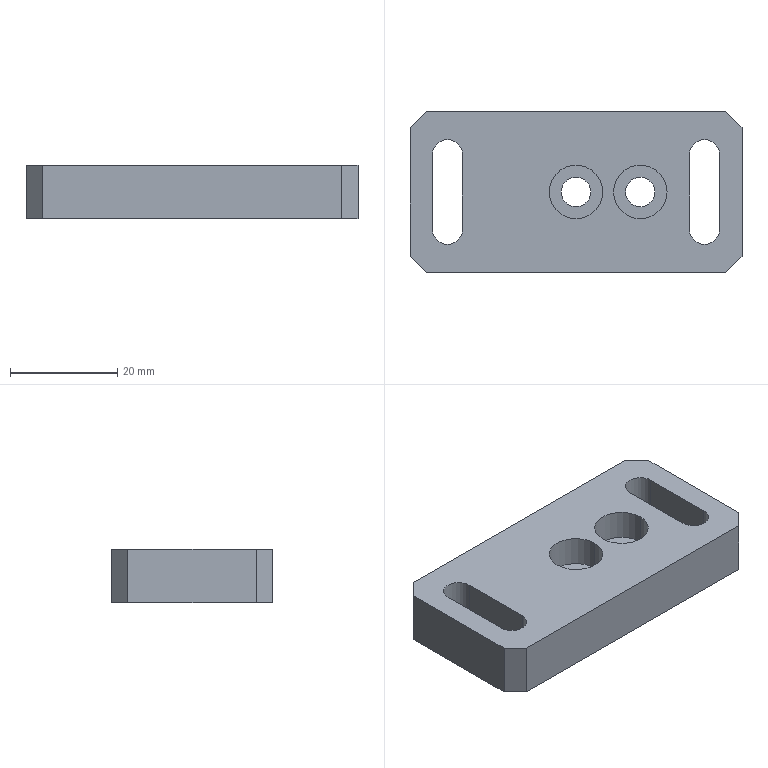Component | SolidWorks | A52-1 | 1 solid | 28 faces | box 62 x 30 x 10 mm | volume 15260 mm3 | plane 16 | cylinder 12 | commonest cylinder face diameters 10 x4 5.5 x4 5.6 x4 | material A6061
build123d program:
from build123d import *

# Parameters (mm, degrees)
SKETCH1_W                                         = 62
SKETCH1_H                                         = 30
BOSS_EXTRUDE1_DEPTH                               = 5
CHAMFER1_SIZE                                     = 3
CUT_EXTRUDE1_DEPTH                                = 36.861
HOLE_SIZE_ACCORDING_TO_HEXAGON_SOCKET_D           = 5.5
HOLE_SIZE_ACCORDING_TO_HEXAGON_SOCKET_CBORE_D     = 10
HOLE_SIZE_ACCORDING_TO_HEXAGON_SOCKET_CBORE_DEPTH = 5.7


with BuildPart() as part:
    # Sketch1 → Boss-Extrude1 (new, symmetric)
    with BuildSketch(Plane(origin=(0, 0, 0), x_dir=(0, 0, -1), z_dir=(1, 0, 0))):
        Rectangle(SKETCH1_W, SKETCH1_H)
    extrude(amount=BOSS_EXTRUDE1_DEPTH, both=True)

    # Chamfer1
    chamfer1_edges = [part.edges().sort_by_distance(p)[0] for p in [
        (0, -15, -31),
        (0, -15, 31),
        (0, 15, 31),
        (0, 15, -31),
    ]]
    chamfer(chamfer1_edges, length=CHAMFER1_SIZE)

    # Sketch2 → Cut-Extrude1 (cut, through all)
    with BuildSketch(Plane.ZY.offset(5)):
        with BuildLine():
            Line((-21.2, 7), (-21.2, -7))
            ThreePointArc((-21.2, -7), (-24, -9.8), (-26.8, -7))
            Line((-26.8, -7), (-26.8, 7))
            ThreePointArc((-26.8, 7), (-24, 9.8), (-21.2, 7))
        make_face()
        with BuildLine():
            Line((26.8, 7), (26.8, -7))
            ThreePointArc((26.8, -7), (24, -9.8), (21.2, -7))
            Line((21.2, -7), (21.2, 7))
            ThreePointArc((21.2, 7), (24, 9.8), (26.8, 7))
        make_face()
    extrude(amount=-CUT_EXTRUDE1_DEPTH, mode=Mode.SUBTRACT)

    # Hole Size _according to_ Hexagon Socket (through all)
    with Locations(Plane(origin=(5, 0, 0), x_dir=(0, 0, -1), z_dir=(1, 0, 0))):
        with Locations((0, 0), (12, 0)):
            CounterBoreHole(HOLE_SIZE_ACCORDING_TO_HEXAGON_SOCKET_D / 2, HOLE_SIZE_ACCORDING_TO_HEXAGON_SOCKET_CBORE_D / 2, HOLE_SIZE_ACCORDING_TO_HEXAGON_SOCKET_CBORE_DEPTH)


solid = part.part

# Placed as in the assembly
solid = solid.moved(Location((-12.351, 25.864, 35), (0, -90, 0)))
STEP:
#1=COLOUR_RGB('',0.7922,0.8196,0.9333);
#2=FILL_AREA_STYLE_COLOUR('',#1);
#3=FILL_AREA_STYLE('',(#2));
#4=SURFACE_STYLE_FILL_AREA(#3);
#5=SURFACE_SIDE_STYLE('',(#4));
#6=SURFACE_STYLE_USAGE(.BOTH.,#5);
#7=PRESENTATION_STYLE_ASSIGNMENT((#6));
#8=CARTESIAN_POINT('',(-0.6831,1.018,1.35));
#9=VERTEX_POINT('',#8);
#10=CARTESIAN_POINT('',(-0.2894,1.018,1.35));
#11=VERTEX_POINT('',#10);
#12=CARTESIAN_POINT('',(-0.4863,1.018,1.35));
#13=DIRECTION('',(0.,0.,1.));
#14=DIRECTION('',(1.,0.,0.));
#15=AXIS2_PLACEMENT_3D('',#12,#13,#14);
#16=CIRCLE('',#15,0.1969);
#17=EDGE_CURVE('',#9,#11,#16,.T.);
#18=ORIENTED_EDGE('',*,*,#17,.F.);
#19=CARTESIAN_POINT('',(-0.6831,1.018,1.575));
#20=VERTEX_POINT('',#19);
#21=CARTESIAN_POINT('',(-0.6831,1.018,1.575));
#22=DIRECTION('',(0.,0.,1.));
#23=VECTOR('',#22,39.37);
#24=LINE('',#21,#23);
#25=EDGE_CURVE('',#9,#20,#24,.T.);
#26=ORIENTED_EDGE('',*,*,#25,.T.);
#27=CARTESIAN_POINT('',(-0.2894,1.018,1.575));
#28=VERTEX_POINT('',#27);
#29=CARTESIAN_POINT('',(-0.4863,1.018,1.575));
#30=DIRECTION('',(0.,0.,1.));
#31=DIRECTION('',(1.,0.,0.));
#32=AXIS2_PLACEMENT_3D('',#29,#30,#31);
#33=CIRCLE('',#32,0.1969);
#34=EDGE_CURVE('',#20,#28,#33,.T.);
#35=ORIENTED_EDGE('',*,*,#34,.T.);
#36=CARTESIAN_POINT('',(-0.2894,1.018,1.575));
#37=DIRECTION('',(0.,0.,1.));
#38=VECTOR('',#37,39.37);
#39=LINE('',#36,#38);
#40=EDGE_CURVE('',#11,#28,#39,.T.);
#41=ORIENTED_EDGE('',*,*,#40,.F.);
#42=EDGE_LOOP('',(#18,#26,#35,#41));
#43=FACE_OUTER_BOUND('',#42,.T.);
#44=CARTESIAN_POINT('',(-0.4863,1.018,1.575));
#45=DIRECTION('',(0.,0.,1.));
#46=DIRECTION('',(1.,0.,0.));
#47=AXIS2_PLACEMENT_3D('',#44,#45,#46);
#48=CYLINDRICAL_SURFACE('',#47,0.1969);
#49=ADVANCED_FACE('',(#43),#48,.F.);
#50=CARTESIAN_POINT('',(-0.5945,1.018,1.181));
#51=VERTEX_POINT('',#50);
#52=CARTESIAN_POINT('',(-0.378,1.018,1.181));
#53=VERTEX_POINT('',#52);
#54=CARTESIAN_POINT('',(-0.4863,1.018,1.181));
#55=DIRECTION('',(0.,0.,1.));
#56=DIRECTION('',(1.,0.,0.));
#57=AXIS2_PLACEMENT_3D('',#54,#55,#56);
#58=CIRCLE('',#57,0.1083);
#59=EDGE_CURVE('',#51,#53,#58,.T.);
#60=ORIENTED_EDGE('',*,*,#59,.F.);
#61=CARTESIAN_POINT('',(-0.5945,1.018,1.35));
#62=VERTEX_POINT('',#61);
#63=CARTESIAN_POINT('',(-0.5945,1.018,1.575));
#64=DIRECTION('',(0.,0.,1.));
#65=VECTOR('',#64,39.37);
#66=LINE('',#63,#65);
#67=EDGE_CURVE('',#51,#62,#66,.T.);
#68=ORIENTED_EDGE('',*,*,#67,.T.);
#69=CARTESIAN_POINT('',(-0.378,1.018,1.35));
#70=VERTEX_POINT('',#69);
#71=CARTESIAN_POINT('',(-0.4863,1.018,1.35));
#72=DIRECTION('',(0.,0.,1.));
#73=DIRECTION('',(1.,0.,0.));
#74=AXIS2_PLACEMENT_3D('',#71,#72,#73);
#75=CIRCLE('',#74,0.1083);
#76=EDGE_CURVE('',#62,#70,#75,.T.);
#77=ORIENTED_EDGE('',*,*,#76,.T.);
#78=CARTESIAN_POINT('',(-0.378,1.018,1.575));
#79=DIRECTION('',(0.,0.,1.));
#80=VECTOR('',#79,39.37);
#81=LINE('',#78,#80);
#82=EDGE_CURVE('',#53,#70,#81,.T.);
#83=ORIENTED_EDGE('',*,*,#82,.F.);
#84=EDGE_LOOP('',(#60,#68,#77,#83));
#85=FACE_OUTER_BOUND('',#84,.T.);
#86=CARTESIAN_POINT('',(-0.4863,1.018,1.575));
#87=DIRECTION('',(0.,0.,1.));
#88=DIRECTION('',(1.,0.,0.));
#89=AXIS2_PLACEMENT_3D('',#86,#87,#88);
#90=CYLINDRICAL_SURFACE('',#89,0.1083);
#91=ADVANCED_FACE('',(#85),#90,.F.);
#92=CARTESIAN_POINT('',(-0.2107,1.018,1.35));
#93=VERTEX_POINT('',#92);
#94=CARTESIAN_POINT('',(0.183,1.018,1.35));
#95=VERTEX_POINT('',#94);
#96=CARTESIAN_POINT('',(-0.01381,1.018,1.35));
#97=DIRECTION('',(0.,0.,1.));
#98=DIRECTION('',(1.,0.,0.));
#99=AXIS2_PLACEMENT_3D('',#96,#97,#98);
#100=CIRCLE('',#99,0.1969);
#101=EDGE_CURVE('',#93,#95,#100,.T.);
#102=ORIENTED_EDGE('',*,*,#101,.F.);
#103=CARTESIAN_POINT('',(-0.2107,1.018,1.575));
#104=VERTEX_POINT('',#103);
#105=CARTESIAN_POINT('',(-0.2107,1.018,1.575));
#106=DIRECTION('',(0.,0.,1.));
#107=VECTOR('',#106,39.37);
#108=LINE('',#105,#107);
#109=EDGE_CURVE('',#93,#104,#108,.T.);
#110=ORIENTED_EDGE('',*,*,#109,.T.);
#111=CARTESIAN_POINT('',(0.183,1.018,1.575));
#112=VERTEX_POINT('',#111);
#113=CARTESIAN_POINT('',(-0.01381,1.018,1.575));
#114=DIRECTION('',(0.,0.,1.));
#115=DIRECTION('',(1.,0.,0.));
#116=AXIS2_PLACEMENT_3D('',#113,#114,#115);
#117=CIRCLE('',#116,0.1969);
#118=EDGE_CURVE('',#104,#112,#117,.T.);
#119=ORIENTED_EDGE('',*,*,#118,.T.);
#120=CARTESIAN_POINT('',(0.183,1.018,1.575));
#121=DIRECTION('',(0.,0.,1.));
#122=VECTOR('',#121,39.37);
#123=LINE('',#120,#122);
#124=EDGE_CURVE('',#95,#112,#123,.T.);
#125=ORIENTED_EDGE('',*,*,#124,.F.);
#126=EDGE_LOOP('',(#102,#110,#119,#125));
#127=FACE_OUTER_BOUND('',#126,.T.);
#128=CARTESIAN_POINT('',(-0.01381,1.018,1.575));
#129=DIRECTION('',(0.,0.,1.));
#130=DIRECTION('',(1.,0.,0.));
#131=AXIS2_PLACEMENT_3D('',#128,#129,#130);
#132=CYLINDRICAL_SURFACE('',#131,0.1969);
#133=ADVANCED_FACE('',(#127),#132,.F.);
#134=CARTESIAN_POINT('',(-0.1221,1.018,1.181));
#135=VERTEX_POINT('',#134);
#136=CARTESIAN_POINT('',(0.09446,1.018,1.181));
#137=VERTEX_POINT('',#136);
#138=CARTESIAN_POINT('',(-0.01381,1.018,1.181));
#139=DIRECTION('',(0.,0.,1.));
#140=DIRECTION('',(1.,0.,0.));
#141=AXIS2_PLACEMENT_3D('',#138,#139,#140);
#142=CIRCLE('',#141,0.1083);
#143=EDGE_CURVE('',#135,#137,#142,.T.);
#144=ORIENTED_EDGE('',*,*,#143,.F.);
#145=CARTESIAN_POINT('',(-0.1221,1.018,1.35));
#146=VERTEX_POINT('',#145);
#147=CARTESIAN_POINT('',(-0.1221,1.018,1.575));
#148=DIRECTION('',(0.,0.,1.));
#149=VECTOR('',#148,39.37);
#150=LINE('',#147,#149);
#151=EDGE_CURVE('',#135,#146,#150,.T.);
#152=ORIENTED_EDGE('',*,*,#151,.T.);
#153=CARTESIAN_POINT('',(0.09446,1.018,1.35));
#154=VERTEX_POINT('',#153);
#155=CARTESIAN_POINT('',(-0.01381,1.018,1.35));
#156=DIRECTION('',(0.,0.,1.));
#157=DIRECTION('',(1.,0.,0.));
#158=AXIS2_PLACEMENT_3D('',#155,#156,#157);
#159=CIRCLE('',#158,0.1083);
#160=EDGE_CURVE('',#146,#154,#159,.T.);
#161=ORIENTED_EDGE('',*,*,#160,.T.);
#162=CARTESIAN_POINT('',(0.09446,1.018,1.575));
#163=DIRECTION('',(0.,0.,1.));
#164=VECTOR('',#163,39.37);
#165=LINE('',#162,#164);
#166=EDGE_CURVE('',#137,#154,#165,.T.);
#167=ORIENTED_EDGE('',*,*,#166,.F.);
#168=EDGE_LOOP('',(#144,#152,#161,#167));
#169=FACE_OUTER_BOUND('',#168,.T.);
#170=CARTESIAN_POINT('',(-0.01381,1.018,1.575));
#171=DIRECTION('',(0.,0.,1.));
#172=DIRECTION('',(1.,0.,0.));
#173=AXIS2_PLACEMENT_3D('',#170,#171,#172);
#174=CYLINDRICAL_SURFACE('',#173,0.1083);
#175=ADVANCED_FACE('',(#169),#174,.F.);
#176=CARTESIAN_POINT('',(0.7342,0.5458,1.181));
#177=VERTEX_POINT('',#176);
#178=CARTESIAN_POINT('',(0.7342,1.491,1.181));
#179=VERTEX_POINT('',#178);
#180=CARTESIAN_POINT('',(0.7342,1.609,1.181));
#181=DIRECTION('',(-0.,1.,0.));
#182=VECTOR('',#181,39.37);
#183=LINE('',#180,#182);
#184=EDGE_CURVE('',#177,#179,#183,.T.);
#185=ORIENTED_EDGE('',*,*,#184,.T.);
#186=CARTESIAN_POINT('',(0.7342,1.491,1.575));
#187=VERTEX_POINT('',#186);
#188=CARTESIAN_POINT('',(0.7342,1.491,1.575));
#189=DIRECTION('',(0.,0.,1.));
#190=VECTOR('',#189,39.37);
#191=LINE('',#188,#190);
#192=EDGE_CURVE('',#179,#187,#191,.T.);
#193=ORIENTED_EDGE('',*,*,#192,.T.);
#194=CARTESIAN_POINT('',(0.7342,0.5458,1.575));
#195=VERTEX_POINT('',#194);
#196=CARTESIAN_POINT('',(0.7342,1.609,1.575));
#197=DIRECTION('',(-0.,1.,0.));
#198=VECTOR('',#197,39.37);
#199=LINE('',#196,#198);
#200=EDGE_CURVE('',#195,#187,#199,.T.);
#201=ORIENTED_EDGE('',*,*,#200,.F.);
#202=CARTESIAN_POINT('',(0.7342,0.5458,1.575));
#203=DIRECTION('',(0.,0.,-1.));
#204=VECTOR('',#203,39.37);
#205=LINE('',#202,#204);
#206=EDGE_CURVE('',#195,#177,#205,.T.);
#207=ORIENTED_EDGE('',*,*,#206,.T.);
#208=EDGE_LOOP('',(#185,#193,#201,#207));
#209=FACE_OUTER_BOUND('',#208,.T.);
#210=CARTESIAN_POINT('',(0.7342,1.609,1.575));
#211=DIRECTION('',(-1.,-0.,0.));
#212=DIRECTION('',(0.,-1.,0.));
#213=AXIS2_PLACEMENT_3D('',#210,#211,#212);
#214=PLANE('',#213);
#215=ADVANCED_FACE('',(#209),#214,.F.);
#216=CARTESIAN_POINT('',(0.6161,1.609,1.575));
#217=VERTEX_POINT('',#216);
#218=CARTESIAN_POINT('',(-1.589,1.609,1.575));
#219=VERTEX_POINT('',#218);
#220=CARTESIAN_POINT('',(-1.707,1.609,1.575));
#221=DIRECTION('',(-1.,0.,0.));
#222=VECTOR('',#221,39.37);
#223=LINE('',#220,#222);
#224=EDGE_CURVE('',#217,#219,#223,.T.);
#225=ORIENTED_EDGE('',*,*,#224,.F.);
#226=CARTESIAN_POINT('',(0.6161,1.609,1.181));
#227=VERTEX_POINT('',#226);
#228=CARTESIAN_POINT('',(0.6161,1.609,1.575));
#229=DIRECTION('',(0.,0.,-1.));
#230=VECTOR('',#229,39.37);
#231=LINE('',#228,#230);
#232=EDGE_CURVE('',#217,#227,#231,.T.);
#233=ORIENTED_EDGE('',*,*,#232,.T.);
#234=CARTESIAN_POINT('',(-1.589,1.609,1.181));
#235=VERTEX_POINT('',#234);
#236=CARTESIAN_POINT('',(-1.707,1.609,1.181));
#237=DIRECTION('',(-1.,0.,0.));
#238=VECTOR('',#237,39.37);
#239=LINE('',#236,#238);
#240=EDGE_CURVE('',#227,#235,#239,.T.);
#241=ORIENTED_EDGE('',*,*,#240,.T.);
#242=CARTESIAN_POINT('',(-1.589,1.609,1.575));
#243=DIRECTION('',(0.,0.,1.));
#244=VECTOR('',#243,39.37);
#245=LINE('',#242,#244);
#246=EDGE_CURVE('',#235,#219,#245,.T.);
#247=ORIENTED_EDGE('',*,*,#246,.T.);
#248=EDGE_LOOP('',(#225,#233,#241,#247));
#249=FACE_OUTER_BOUND('',#248,.T.);
#250=CARTESIAN_POINT('',(-1.707,1.609,1.575));
#251=DIRECTION('',(0.,-1.,0.));
#252=DIRECTION('',(1.,0.,0.));
#253=AXIS2_PLACEMENT_3D('',#250,#251,#252);
#254=PLANE('',#253);
#255=ADVANCED_FACE('',(#249),#254,.F.);
#256=CARTESIAN_POINT('',(-1.707,1.491,1.181));
#257=VERTEX_POINT('',#256);
#258=CARTESIAN_POINT('',(-1.707,0.5458,1.181));
#259=VERTEX_POINT('',#258);
#260=CARTESIAN_POINT('',(-1.707,1.609,1.181));
#261=DIRECTION('',(0.,-1.,0.));
#262=VECTOR('',#261,39.37);
#263=LINE('',#260,#262);
#264=EDGE_CURVE('',#257,#259,#263,.T.);
#265=ORIENTED_EDGE('',*,*,#264,.T.);
#266=CARTESIAN_POINT('',(-1.707,0.5458,1.575));
#267=VERTEX_POINT('',#266);
#268=CARTESIAN_POINT('',(-1.707,0.5458,1.575));
#269=DIRECTION('',(0.,0.,1.));
#270=VECTOR('',#269,39.37);
#271=LINE('',#268,#270);
#272=EDGE_CURVE('',#259,#267,#271,.T.);
#273=ORIENTED_EDGE('',*,*,#272,.T.);
#274=CARTESIAN_POINT('',(-1.707,1.491,1.575));
#275=VERTEX_POINT('',#274);
#276=CARTESIAN_POINT('',(-1.707,1.609,1.575));
#277=DIRECTION('',(0.,-1.,0.));
#278=VECTOR('',#277,39.37);
#279=LINE('',#276,#278);
#280=EDGE_CURVE('',#275,#267,#279,.T.);
#281=ORIENTED_EDGE('',*,*,#280,.F.);
#282=CARTESIAN_POINT('',(-1.707,1.491,1.575));
#283=DIRECTION('',(0.,0.,-1.));
#284=VECTOR('',#283,39.37);
#285=LINE('',#282,#284);
#286=EDGE_CURVE('',#275,#257,#285,.T.);
#287=ORIENTED_EDGE('',*,*,#286,.T.);
#288=EDGE_LOOP('',(#265,#273,#281,#287));
#289=FACE_OUTER_BOUND('',#288,.T.);
#290=CARTESIAN_POINT('',(-1.707,1.609,1.575));
#291=DIRECTION('',(1.,0.,0.));
#292=DIRECTION('',(0.,0.,-1.));
#293=AXIS2_PLACEMENT_3D('',#290,#291,#292);
#294=PLANE('',#293);
#295=ADVANCED_FACE('',(#289),#294,.F.);
#296=CARTESIAN_POINT('',(-1.589,0.4277,1.181));
#297=VERTEX_POINT('',#296);
#298=CARTESIAN_POINT('',(0.6161,0.4277,1.181));
#299=VERTEX_POINT('',#298);
#300=CARTESIAN_POINT('',(-1.707,0.4277,1.181));
#301=DIRECTION('',(1.,0.,0.));
#302=VECTOR('',#301,39.37);
#303=LINE('',#300,#302);
#304=EDGE_CURVE('',#297,#299,#303,.T.);
#305=ORIENTED_EDGE('',*,*,#304,.T.);
#306=CARTESIAN_POINT('',(0.6161,0.4277,1.575));
#307=VERTEX_POINT('',#306);
#308=CARTESIAN_POINT('',(0.6161,0.4277,1.575));
#309=DIRECTION('',(0.,0.,1.));
#310=VECTOR('',#309,39.37);
#311=LINE('',#308,#310);
#312=EDGE_CURVE('',#299,#307,#311,.T.);
#313=ORIENTED_EDGE('',*,*,#312,.T.);
#314=CARTESIAN_POINT('',(-1.589,0.4277,1.575));
#315=VERTEX_POINT('',#314);
#316=CARTESIAN_POINT('',(-1.707,0.4277,1.575));
#317=DIRECTION('',(1.,0.,0.));
#318=VECTOR('',#317,39.37);
#319=LINE('',#316,#318);
#320=EDGE_CURVE('',#315,#307,#319,.T.);
#321=ORIENTED_EDGE('',*,*,#320,.F.);
#322=CARTESIAN_POINT('',(-1.589,0.4277,1.575));
#323=DIRECTION('',(0.,0.,-1.));
#324=VECTOR('',#323,39.37);
#325=LINE('',#322,#324);
#326=EDGE_CURVE('',#315,#297,#325,.T.);
#327=ORIENTED_EDGE('',*,*,#326,.T.);
#328=EDGE_LOOP('',(#305,#313,#321,#327));
#329=FACE_OUTER_BOUND('',#328,.T.);
#330=CARTESIAN_POINT('',(-1.707,0.4277,1.575));
#331=DIRECTION('',(0.,1.,0.));
#332=DIRECTION('',(-1.,0.,0.));
#333=AXIS2_PLACEMENT_3D('',#330,#331,#332);
#334=PLANE('',#333);
#335=ADVANCED_FACE('',(#329),#334,.F.);
#336=CARTESIAN_POINT('',(-0.4863,1.018,1.575));
#337=DIRECTION('',(0.,0.,1.));
#338=DIRECTION('',(1.,0.,0.));
#339=AXIS2_PLACEMENT_3D('',#336,#337,#338);
#340=CIRCLE('',#339,0.1969);
#341=EDGE_CURVE('',#28,#20,#340,.T.);
#342=ORIENTED_EDGE('',*,*,#341,.F.);
#343=ORIENTED_EDGE('',*,*,#34,.F.);
#344=EDGE_LOOP('',(#342,#343));
#345=FACE_BOUND('',#344,.T.);
#346=CARTESIAN_POINT('',(-0.01381,1.018,1.575));
#347=DIRECTION('',(0.,0.,1.));
#348=DIRECTION('',(1.,0.,0.));
#349=AXIS2_PLACEMENT_3D('',#346,#347,#348);
#350=CIRCLE('',#349,0.1969);
#351=EDGE_CURVE('',#112,#104,#350,.T.);
#352=ORIENTED_EDGE('',*,*,#351,.F.);
#353=ORIENTED_EDGE('',*,*,#118,.F.);
#354=EDGE_LOOP('',(#352,#353));
#355=FACE_BOUND('',#354,.T.);
#356=CARTESIAN_POINT('',(0.3484,1.294,1.575));
#357=VERTEX_POINT('',#356);
#358=CARTESIAN_POINT('',(0.5689,1.294,1.575));
#359=VERTEX_POINT('',#358);
#360=CARTESIAN_POINT('',(0.4586,1.294,1.575));
#361=DIRECTION('',(0.,0.,-1.));
#362=DIRECTION('',(-1.,0.,0.));
#363=AXIS2_PLACEMENT_3D('',#360,#361,#362);
#364=CIRCLE('',#363,0.1102);
#365=EDGE_CURVE('',#357,#359,#364,.T.);
#366=ORIENTED_EDGE('',*,*,#365,.T.);
#367=CARTESIAN_POINT('',(0.5689,0.7427,1.575));
#368=VERTEX_POINT('',#367);
#369=CARTESIAN_POINT('',(0.5689,1.294,1.575));
#370=DIRECTION('',(0.,-1.,0.));
#371=VECTOR('',#370,39.37);
#372=LINE('',#369,#371);
#373=EDGE_CURVE('',#359,#368,#372,.T.);
#374=ORIENTED_EDGE('',*,*,#373,.T.);
#375=CARTESIAN_POINT('',(0.3484,0.7427,1.575));
#376=VERTEX_POINT('',#375);
#377=CARTESIAN_POINT('',(0.4586,0.7427,1.575));
#378=DIRECTION('',(0.,0.,-1.));
#379=DIRECTION('',(-1.,0.,0.));
#380=AXIS2_PLACEMENT_3D('',#377,#378,#379);
#381=CIRCLE('',#380,0.1102);
#382=EDGE_CURVE('',#368,#376,#381,.T.);
#383=ORIENTED_EDGE('',*,*,#382,.T.);
#384=CARTESIAN_POINT('',(0.3484,1.294,1.575));
#385=DIRECTION('',(0.,1.,0.));
#386=VECTOR('',#385,39.37);
#387=LINE('',#384,#386);
#388=EDGE_CURVE('',#376,#357,#387,.T.);
#389=ORIENTED_EDGE('',*,*,#388,.T.);
#390=EDGE_LOOP('',(#366,#374,#383,#389));
#391=FACE_BOUND('',#390,.T.);
#392=CARTESIAN_POINT('',(-1.541,1.294,1.575));
#393=VERTEX_POINT('',#392);
#394=CARTESIAN_POINT('',(-1.321,1.294,1.575));
#395=VERTEX_POINT('',#394);
#396=CARTESIAN_POINT('',(-1.431,1.294,1.575));
#397=DIRECTION('',(0.,0.,-1.));
#398=DIRECTION('',(-1.,0.,0.));
#399=AXIS2_PLACEMENT_3D('',#396,#397,#398);
#400=CIRCLE('',#399,0.1102);
#401=EDGE_CURVE('',#393,#395,#400,.T.);
#402=ORIENTED_EDGE('',*,*,#401,.T.);
#403=CARTESIAN_POINT('',(-1.321,0.7427,1.575));
#404=VERTEX_POINT('',#403);
#405=CARTESIAN_POINT('',(-1.321,1.294,1.575));
#406=DIRECTION('',(0.,-1.,0.));
#407=VECTOR('',#406,39.37);
#408=LINE('',#405,#407);
#409=EDGE_CURVE('',#395,#404,#408,.T.);
#410=ORIENTED_EDGE('',*,*,#409,.T.);
#411=CARTESIAN_POINT('',(-1.541,0.7427,1.575));
#412=VERTEX_POINT('',#411);
#413=CARTESIAN_POINT('',(-1.431,0.7427,1.575));
#414=DIRECTION('',(0.,0.,-1.));
#415=DIRECTION('',(-1.,0.,0.));
#416=AXIS2_PLACEMENT_3D('',#413,#414,#415);
#417=CIRCLE('',#416,0.1102);
#418=EDGE_CURVE('',#404,#412,#417,.T.);
#419=ORIENTED_EDGE('',*,*,#418,.T.);
#420=CARTESIAN_POINT('',(-1.541,1.294,1.575));
#421=DIRECTION('',(0.,1.,0.));
#422=VECTOR('',#421,39.37);
#423=LINE('',#420,#422);
#424=EDGE_CURVE('',#412,#393,#423,.T.);
#425=ORIENTED_EDGE('',*,*,#424,.T.);
#426=EDGE_LOOP('',(#402,#410,#419,#425));
#427=FACE_BOUND('',#426,.T.);
#428=ORIENTED_EDGE('',*,*,#200,.T.);
#429=CARTESIAN_POINT('',(0.3602,1.865,1.575));
#430=DIRECTION('',(-0.7071,0.7071,0.));
#431=VECTOR('',#430,39.37);
#432=LINE('',#429,#431);
#433=EDGE_CURVE('',#187,#217,#432,.T.);
#434=ORIENTED_EDGE('',*,*,#433,.T.);
#435=ORIENTED_EDGE('',*,*,#224,.T.);
#436=CARTESIAN_POINT('',(-1.333,1.865,1.575));
#437=DIRECTION('',(-0.7071,-0.7071,0.));
#438=VECTOR('',#437,39.37);
#439=LINE('',#436,#438);
#440=EDGE_CURVE('',#219,#275,#439,.T.);
#441=ORIENTED_EDGE('',*,*,#440,.T.);
#442=ORIENTED_EDGE('',*,*,#280,.T.);
#443=CARTESIAN_POINT('',(-1.333,0.1718,1.575));
#444=DIRECTION('',(0.7071,-0.7071,0.));
#445=VECTOR('',#444,39.37);
#446=LINE('',#443,#445);
#447=EDGE_CURVE('',#267,#315,#446,.T.);
#448=ORIENTED_EDGE('',*,*,#447,.T.);
#449=ORIENTED_EDGE('',*,*,#320,.T.);
#450=CARTESIAN_POINT('',(0.3602,0.1718,1.575));
#451=DIRECTION('',(0.7071,0.7071,0.));
#452=VECTOR('',#451,39.37);
#453=LINE('',#450,#452);
#454=EDGE_CURVE('',#307,#195,#453,.T.);
#455=ORIENTED_EDGE('',*,*,#454,.T.);
#456=EDGE_LOOP('',(#428,#434,#435,#441,#442,#448,#449,#455));
#457=FACE_OUTER_BOUND('',#456,.T.);
#458=CARTESIAN_POINT('',(-0.4863,1.018,1.575));
#459=DIRECTION('',(0.,0.,1.));
#460=DIRECTION('',(1.,0.,0.));
#461=AXIS2_PLACEMENT_3D('',#458,#459,#460);
#462=PLANE('',#461);
#463=ADVANCED_FACE('',(#345,#355,#391,#427,#457),#462,.T.);
#464=CARTESIAN_POINT('',(-0.4863,1.018,1.181));
#465=DIRECTION('',(0.,0.,1.));
#466=DIRECTION('',(1.,0.,0.));
#467=AXIS2_PLACEMENT_3D('',#464,#465,#466);
#468=CIRCLE('',#467,0.1083);
#469=EDGE_CURVE('',#53,#51,#468,.T.);
#470=ORIENTED_EDGE('',*,*,#469,.T.);
#471=ORIENTED_EDGE('',*,*,#59,.T.);
#472=EDGE_LOOP('',(#470,#471));
#473=FACE_BOUND('',#472,.T.);
#474=CARTESIAN_POINT('',(-0.01381,1.018,1.181));
#475=DIRECTION('',(0.,0.,1.));
#476=DIRECTION('',(1.,0.,0.));
#477=AXIS2_PLACEMENT_3D('',#474,#475,#476);
#478=CIRCLE('',#477,0.1083);
#479=EDGE_CURVE('',#137,#135,#478,.T.);
#480=ORIENTED_EDGE('',*,*,#479,.T.);
#481=ORIENTED_EDGE('',*,*,#143,.T.);
#482=EDGE_LOOP('',(#480,#481));
#483=FACE_BOUND('',#482,.T.);
#484=CARTESIAN_POINT('',(0.5689,1.294,1.181));
#485=VERTEX_POINT('',#484);
#486=CARTESIAN_POINT('',(0.5689,0.7427,1.181));
#487=VERTEX_POINT('',#486);
#488=CARTESIAN_POINT('',(0.5689,1.294,1.181));
#489=DIRECTION('',(0.,-1.,0.));
#490=VECTOR('',#489,39.37);
#491=LINE('',#488,#490);
#492=EDGE_CURVE('',#485,#487,#491,.T.);
#493=ORIENTED_EDGE('',*,*,#492,.F.);
#494=CARTESIAN_POINT('',(0.3484,1.294,1.181));
#495=VERTEX_POINT('',#494);
#496=CARTESIAN_POINT('',(0.4586,1.294,1.181));
#497=DIRECTION('',(0.,0.,-1.));
#498=DIRECTION('',(-1.,0.,0.));
#499=AXIS2_PLACEMENT_3D('',#496,#497,#498);
#500=CIRCLE('',#499,0.1102);
#501=EDGE_CURVE('',#495,#485,#500,.T.);
#502=ORIENTED_EDGE('',*,*,#501,.F.);
#503=CARTESIAN_POINT('',(0.3484,0.7427,1.181));
#504=VERTEX_POINT('',#503);
#505=CARTESIAN_POINT('',(0.3484,1.294,1.181));
#506=DIRECTION('',(0.,1.,0.));
#507=VECTOR('',#506,39.37);
#508=LINE('',#505,#507);
#509=EDGE_CURVE('',#504,#495,#508,.T.);
#510=ORIENTED_EDGE('',*,*,#509,.F.);
#511=CARTESIAN_POINT('',(0.4586,0.7427,1.181));
#512=DIRECTION('',(0.,0.,-1.));
#513=DIRECTION('',(-1.,0.,0.));
#514=AXIS2_PLACEMENT_3D('',#511,#512,#513);
#515=CIRCLE('',#514,0.1102);
#516=EDGE_CURVE('',#487,#504,#515,.T.);
#517=ORIENTED_EDGE('',*,*,#516,.F.);
#518=EDGE_LOOP('',(#493,#502,#510,#517));
#519=FACE_BOUND('',#518,.T.);
#520=CARTESIAN_POINT('',(-1.321,1.294,1.181));
#521=VERTEX_POINT('',#520);
#522=CARTESIAN_POINT('',(-1.321,0.7427,1.181));
#523=VERTEX_POINT('',#522);
#524=CARTESIAN_POINT('',(-1.321,1.294,1.181));
#525=DIRECTION('',(0.,-1.,0.));
#526=VECTOR('',#525,39.37);
#527=LINE('',#524,#526);
#528=EDGE_CURVE('',#521,#523,#527,.T.);
#529=ORIENTED_EDGE('',*,*,#528,.F.);
#530=CARTESIAN_POINT('',(-1.541,1.294,1.181));
#531=VERTEX_POINT('',#530);
#532=CARTESIAN_POINT('',(-1.431,1.294,1.181));
#533=DIRECTION('',(0.,0.,-1.));
#534=DIRECTION('',(-1.,0.,0.));
#535=AXIS2_PLACEMENT_3D('',#532,#533,#534);
#536=CIRCLE('',#535,0.1102);
#537=EDGE_CURVE('',#531,#521,#536,.T.);
#538=ORIENTED_EDGE('',*,*,#537,.F.);
#539=CARTESIAN_POINT('',(-1.541,0.7427,1.181));
#540=VERTEX_POINT('',#539);
#541=CARTESIAN_POINT('',(-1.541,1.294,1.181));
#542=DIRECTION('',(0.,1.,0.));
#543=VECTOR('',#542,39.37);
#544=LINE('',#541,#543);
#545=EDGE_CURVE('',#540,#531,#544,.T.);
#546=ORIENTED_EDGE('',*,*,#545,.F.);
#547=CARTESIAN_POINT('',(-1.431,0.7427,1.181));
#548=DIRECTION('',(0.,0.,-1.));
#549=DIRECTION('',(-1.,0.,0.));
#550=AXIS2_PLACEMENT_3D('',#547,#548,#549);
#551=CIRCLE('',#550,0.1102);
#552=EDGE_CURVE('',#523,#540,#551,.T.);
#553=ORIENTED_EDGE('',*,*,#552,.F.);
#554=EDGE_LOOP('',(#529,#538,#546,#553));
#555=FACE_BOUND('',#554,.T.);
#556=ORIENTED_EDGE('',*,*,#240,.F.);
#557=CARTESIAN_POINT('',(0.6161,1.609,1.181));
#558=DIRECTION('',(0.7071,-0.7071,0.));
#559=VECTOR('',#558,39.37);
#560=LINE('',#557,#559);
#561=EDGE_CURVE('',#227,#179,#560,.T.);
#562=ORIENTED_EDGE('',*,*,#561,.T.);
#563=ORIENTED_EDGE('',*,*,#184,.F.);
#564=CARTESIAN_POINT('',(0.7342,0.5458,1.181));
#565=DIRECTION('',(-0.7071,-0.7071,0.));
#566=VECTOR('',#565,39.37);
#567=LINE('',#564,#566);
#568=EDGE_CURVE('',#177,#299,#567,.T.);
#569=ORIENTED_EDGE('',*,*,#568,.T.);
#570=ORIENTED_EDGE('',*,*,#304,.F.);
#571=CARTESIAN_POINT('',(-1.589,0.4277,1.181));
#572=DIRECTION('',(-0.7071,0.7071,0.));
#573=VECTOR('',#572,39.37);
#574=LINE('',#571,#573);
#575=EDGE_CURVE('',#297,#259,#574,.T.);
#576=ORIENTED_EDGE('',*,*,#575,.T.);
#577=ORIENTED_EDGE('',*,*,#264,.F.);
#578=CARTESIAN_POINT('',(-1.707,1.491,1.181));
#579=DIRECTION('',(0.7071,0.7071,0.));
#580=VECTOR('',#579,39.37);
#581=LINE('',#578,#580);
#582=EDGE_CURVE('',#257,#235,#581,.T.);
#583=ORIENTED_EDGE('',*,*,#582,.T.);
#584=EDGE_LOOP('',(#556,#562,#563,#569,#570,#576,#577,#583));
#585=FACE_OUTER_BOUND('',#584,.T.);
#586=CARTESIAN_POINT('',(-0.4863,1.018,1.181));
#587=DIRECTION('',(0.,0.,1.));
#588=DIRECTION('',(1.,0.,0.));
#589=AXIS2_PLACEMENT_3D('',#586,#587,#588);
#590=PLANE('',#589);
#591=ADVANCED_FACE('',(#473,#483,#519,#555,#585),#590,.F.);
#592=ORIENTED_EDGE('',*,*,#433,.F.);
#593=ORIENTED_EDGE('',*,*,#192,.F.);
#594=ORIENTED_EDGE('',*,*,#561,.F.);
#595=ORIENTED_EDGE('',*,*,#232,.F.);
#596=EDGE_LOOP('',(#592,#593,#594,#595));
#597=FACE_OUTER_BOUND('',#596,.T.);
#598=CARTESIAN_POINT('',(0.6161,1.609,1.575));
#599=DIRECTION('',(-0.7071,-0.7071,0.));
#600=DIRECTION('',(0.,0.,-1.));
#601=AXIS2_PLACEMENT_3D('',#598,#599,#600);
#602=PLANE('',#601);
#603=ADVANCED_FACE('',(#597),#602,.F.);
#604=ORIENTED_EDGE('',*,*,#454,.F.);
#605=ORIENTED_EDGE('',*,*,#312,.F.);
#606=ORIENTED_EDGE('',*,*,#568,.F.);
#607=ORIENTED_EDGE('',*,*,#206,.F.);
#608=EDGE_LOOP('',(#604,#605,#606,#607));
#609=FACE_OUTER_BOUND('',#608,.T.);
#610=CARTESIAN_POINT('',(0.7342,0.5458,1.575));
#611=DIRECTION('',(-0.7071,0.7071,0.));
#612=DIRECTION('',(0.,0.,-1.));
#613=AXIS2_PLACEMENT_3D('',#610,#611,#612);
#614=PLANE('',#613);
#615=ADVANCED_FACE('',(#609),#614,.F.);
#616=ORIENTED_EDGE('',*,*,#447,.F.);
#617=ORIENTED_EDGE('',*,*,#272,.F.);
#618=ORIENTED_EDGE('',*,*,#575,.F.);
#619=ORIENTED_EDGE('',*,*,#326,.F.);
#620=EDGE_LOOP('',(#616,#617,#618,#619));
#621=FACE_OUTER_BOUND('',#620,.T.);
#622=CARTESIAN_POINT('',(-1.589,0.4277,1.575));
#623=DIRECTION('',(0.7071,0.7071,0.));
#624=DIRECTION('',(0.,0.,-1.));
#625=AXIS2_PLACEMENT_3D('',#622,#623,#624);
#626=PLANE('',#625);
#627=ADVANCED_FACE('',(#621),#626,.F.);
#628=ORIENTED_EDGE('',*,*,#440,.F.);
#629=ORIENTED_EDGE('',*,*,#246,.F.);
#630=ORIENTED_EDGE('',*,*,#582,.F.);
#631=ORIENTED_EDGE('',*,*,#286,.F.);
#632=EDGE_LOOP('',(#628,#629,#630,#631));
#633=FACE_OUTER_BOUND('',#632,.T.);
#634=CARTESIAN_POINT('',(-1.707,1.491,1.575));
#635=DIRECTION('',(0.7071,-0.7071,0.));
#636=DIRECTION('',(0.,0.,-1.));
#637=AXIS2_PLACEMENT_3D('',#634,#635,#636);
#638=PLANE('',#637);
#639=ADVANCED_FACE('',(#633),#638,.F.);
#640=ORIENTED_EDGE('',*,*,#537,.T.);
#641=CARTESIAN_POINT('',(-1.321,1.294,1.575));
#642=DIRECTION('',(0.,0.,-1.));
#643=VECTOR('',#642,39.37);
#644=LINE('',#641,#643);
#645=EDGE_CURVE('',#395,#521,#644,.T.);
#646=ORIENTED_EDGE('',*,*,#645,.F.);
#647=ORIENTED_EDGE('',*,*,#401,.F.);
#648=CARTESIAN_POINT('',(-1.541,1.294,1.575));
#649=DIRECTION('',(0.,0.,-1.));
#650=VECTOR('',#649,39.37);
#651=LINE('',#648,#650);
#652=EDGE_CURVE('',#393,#531,#651,.T.);
#653=ORIENTED_EDGE('',*,*,#652,.T.);
#654=EDGE_LOOP('',(#640,#646,#647,#653));
#655=FACE_OUTER_BOUND('',#654,.T.);
#656=CARTESIAN_POINT('',(-1.431,1.294,1.575));
#657=DIRECTION('',(0.,0.,-1.));
#658=DIRECTION('',(-1.,0.,0.));
#659=AXIS2_PLACEMENT_3D('',#656,#657,#658);
#660=CYLINDRICAL_SURFACE('',#659,0.1102);
#661=ADVANCED_FACE('',(#655),#660,.F.);
#662=ORIENTED_EDGE('',*,*,#545,.T.);
#663=ORIENTED_EDGE('',*,*,#652,.F.);
#664=ORIENTED_EDGE('',*,*,#424,.F.);
#665=CARTESIAN_POINT('',(-1.541,0.7427,1.575));
#666=DIRECTION('',(0.,0.,-1.));
#667=VECTOR('',#666,39.37);
#668=LINE('',#665,#667);
#669=EDGE_CURVE('',#412,#540,#668,.T.);
#670=ORIENTED_EDGE('',*,*,#669,.T.);
#671=EDGE_LOOP('',(#662,#663,#664,#670));
#672=FACE_OUTER_BOUND('',#671,.T.);
#673=CARTESIAN_POINT('',(-1.541,1.294,1.575));
#674=DIRECTION('',(-1.,0.,0.));
#675=DIRECTION('',(0.,0.,1.));
#676=AXIS2_PLACEMENT_3D('',#673,#674,#675);
#677=PLANE('',#676);
#678=ADVANCED_FACE('',(#672),#677,.F.);
#679=ORIENTED_EDGE('',*,*,#552,.T.);
#680=ORIENTED_EDGE('',*,*,#669,.F.);
#681=ORIENTED_EDGE('',*,*,#418,.F.);
#682=CARTESIAN_POINT('',(-1.321,0.7427,1.575));
#683=DIRECTION('',(0.,0.,-1.));
#684=VECTOR('',#683,39.37);
#685=LINE('',#682,#684);
#686=EDGE_CURVE('',#404,#523,#685,.T.);
#687=ORIENTED_EDGE('',*,*,#686,.T.);
#688=EDGE_LOOP('',(#679,#680,#681,#687));
#689=FACE_OUTER_BOUND('',#688,.T.);
#690=CARTESIAN_POINT('',(-1.431,0.7427,1.575));
#691=DIRECTION('',(0.,0.,-1.));
#692=DIRECTION('',(-1.,0.,0.));
#693=AXIS2_PLACEMENT_3D('',#690,#691,#692);
#694=CYLINDRICAL_SURFACE('',#693,0.1102);
#695=ADVANCED_FACE('',(#689),#694,.F.);
#696=ORIENTED_EDGE('',*,*,#528,.T.);
#697=ORIENTED_EDGE('',*,*,#686,.F.);
#698=ORIENTED_EDGE('',*,*,#409,.F.);
#699=ORIENTED_EDGE('',*,*,#645,.T.);
#700=EDGE_LOOP('',(#696,#697,#698,#699));
#701=FACE_OUTER_BOUND('',#700,.T.);
#702=CARTESIAN_POINT('',(-1.321,1.294,1.575));
#703=DIRECTION('',(1.,0.,0.));
#704=DIRECTION('',(0.,0.,-1.));
#705=AXIS2_PLACEMENT_3D('',#702,#703,#704);
#706=PLANE('',#705);
#707=ADVANCED_FACE('',(#701),#706,.F.);
#708=ORIENTED_EDGE('',*,*,#501,.T.);
#709=CARTESIAN_POINT('',(0.5689,1.294,1.575));
#710=DIRECTION('',(0.,0.,-1.));
#711=VECTOR('',#710,39.37);
#712=LINE('',#709,#711);
#713=EDGE_CURVE('',#359,#485,#712,.T.);
#714=ORIENTED_EDGE('',*,*,#713,.F.);
#715=ORIENTED_EDGE('',*,*,#365,.F.);
#716=CARTESIAN_POINT('',(0.3484,1.294,1.575));
#717=DIRECTION('',(0.,0.,-1.));
#718=VECTOR('',#717,39.37);
#719=LINE('',#716,#718);
#720=EDGE_CURVE('',#357,#495,#719,.T.);
#721=ORIENTED_EDGE('',*,*,#720,.T.);
#722=EDGE_LOOP('',(#708,#714,#715,#721));
#723=FACE_OUTER_BOUND('',#722,.T.);
#724=CARTESIAN_POINT('',(0.4586,1.294,1.575));
#725=DIRECTION('',(0.,0.,-1.));
#726=DIRECTION('',(-1.,0.,0.));
#727=AXIS2_PLACEMENT_3D('',#724,#725,#726);
#728=CYLINDRICAL_SURFACE('',#727,0.1102);
#729=ADVANCED_FACE('',(#723),#728,.F.);
#730=ORIENTED_EDGE('',*,*,#509,.T.);
#731=ORIENTED_EDGE('',*,*,#720,.F.);
#732=ORIENTED_EDGE('',*,*,#388,.F.);
#733=CARTESIAN_POINT('',(0.3484,0.7427,1.575));
#734=DIRECTION('',(0.,0.,-1.));
#735=VECTOR('',#734,39.37);
#736=LINE('',#733,#735);
#737=EDGE_CURVE('',#376,#504,#736,.T.);
#738=ORIENTED_EDGE('',*,*,#737,.T.);
#739=EDGE_LOOP('',(#730,#731,#732,#738));
#740=FACE_OUTER_BOUND('',#739,.T.);
#741=CARTESIAN_POINT('',(0.3484,1.294,1.575));
#742=DIRECTION('',(-1.,0.,0.));
#743=DIRECTION('',(-0.,-1.,0.));
#744=AXIS2_PLACEMENT_3D('',#741,#742,#743);
#745=PLANE('',#744);
#746=ADVANCED_FACE('',(#740),#745,.F.);
#747=ORIENTED_EDGE('',*,*,#516,.T.);
#748=ORIENTED_EDGE('',*,*,#737,.F.);
#749=ORIENTED_EDGE('',*,*,#382,.F.);
#750=CARTESIAN_POINT('',(0.5689,0.7427,1.575));
#751=DIRECTION('',(0.,0.,-1.));
#752=VECTOR('',#751,39.37);
#753=LINE('',#750,#752);
#754=EDGE_CURVE('',#368,#487,#753,.T.);
#755=ORIENTED_EDGE('',*,*,#754,.T.);
#756=EDGE_LOOP('',(#747,#748,#749,#755));
#757=FACE_OUTER_BOUND('',#756,.T.);
#758=CARTESIAN_POINT('',(0.4586,0.7427,1.575));
#759=DIRECTION('',(0.,0.,-1.));
#760=DIRECTION('',(-1.,0.,0.));
#761=AXIS2_PLACEMENT_3D('',#758,#759,#760);
#762=CYLINDRICAL_SURFACE('',#761,0.1102);
#763=ADVANCED_FACE('',(#757),#762,.F.);
#764=ORIENTED_EDGE('',*,*,#492,.T.);
#765=ORIENTED_EDGE('',*,*,#754,.F.);
#766=ORIENTED_EDGE('',*,*,#373,.F.);
#767=ORIENTED_EDGE('',*,*,#713,.T.);
#768=EDGE_LOOP('',(#764,#765,#766,#767));
#769=FACE_OUTER_BOUND('',#768,.T.);
#770=CARTESIAN_POINT('',(0.5689,1.294,1.575));
#771=DIRECTION('',(1.,0.,0.));
#772=DIRECTION('',(0.,0.,-1.));
#773=AXIS2_PLACEMENT_3D('',#770,#771,#772);
#774=PLANE('',#773);
#775=ADVANCED_FACE('',(#769),#774,.F.);
#776=ORIENTED_EDGE('',*,*,#151,.F.);
#777=ORIENTED_EDGE('',*,*,#479,.F.);
#778=ORIENTED_EDGE('',*,*,#166,.T.);
#779=CARTESIAN_POINT('',(-0.01381,1.018,1.35));
#780=DIRECTION('',(0.,0.,1.));
#781=DIRECTION('',(1.,0.,0.));
#782=AXIS2_PLACEMENT_3D('',#779,#780,#781);
#783=CIRCLE('',#782,0.1083);
#784=EDGE_CURVE('',#154,#146,#783,.T.);
#785=ORIENTED_EDGE('',*,*,#784,.T.);
#786=EDGE_LOOP('',(#776,#777,#778,#785));
#787=FACE_OUTER_BOUND('',#786,.T.);
#788=CARTESIAN_POINT('',(-0.01381,1.018,1.575));
#789=DIRECTION('',(0.,0.,1.));
#790=DIRECTION('',(1.,0.,0.));
#791=AXIS2_PLACEMENT_3D('',#788,#789,#790);
#792=CYLINDRICAL_SURFACE('',#791,0.1083);
#793=ADVANCED_FACE('',(#787),#792,.F.);
#794=ORIENTED_EDGE('',*,*,#784,.F.);
#795=ORIENTED_EDGE('',*,*,#160,.F.);
#796=EDGE_LOOP('',(#794,#795));
#797=FACE_BOUND('',#796,.T.);
#798=CARTESIAN_POINT('',(-0.01381,1.018,1.35));
#799=DIRECTION('',(0.,0.,1.));
#800=DIRECTION('',(1.,0.,0.));
#801=AXIS2_PLACEMENT_3D('',#798,#799,#800);
#802=CIRCLE('',#801,0.1969);
#803=EDGE_CURVE('',#95,#93,#802,.T.);
#804=ORIENTED_EDGE('',*,*,#803,.T.);
#805=ORIENTED_EDGE('',*,*,#101,.T.);
#806=EDGE_LOOP('',(#804,#805));
#807=FACE_OUTER_BOUND('',#806,.T.);
#808=CARTESIAN_POINT('',(-0.01381,1.127,1.35));
#809=DIRECTION('',(0.,0.,-1.));
#810=DIRECTION('',(-1.,0.,0.));
#811=AXIS2_PLACEMENT_3D('',#808,#809,#810);
#812=PLANE('',#811);
#813=ADVANCED_FACE('',(#797,#807),#812,.F.);
#814=ORIENTED_EDGE('',*,*,#109,.F.);
#815=ORIENTED_EDGE('',*,*,#803,.F.);
#816=ORIENTED_EDGE('',*,*,#124,.T.);
#817=ORIENTED_EDGE('',*,*,#351,.T.);
#818=EDGE_LOOP('',(#814,#815,#816,#817));
#819=FACE_OUTER_BOUND('',#818,.T.);
#820=CARTESIAN_POINT('',(-0.01381,1.018,1.575));
#821=DIRECTION('',(0.,0.,1.));
#822=DIRECTION('',(1.,0.,0.));
#823=AXIS2_PLACEMENT_3D('',#820,#821,#822);
#824=CYLINDRICAL_SURFACE('',#823,0.1969);
#825=ADVANCED_FACE('',(#819),#824,.F.);
#826=ORIENTED_EDGE('',*,*,#67,.F.);
#827=ORIENTED_EDGE('',*,*,#469,.F.);
#828=ORIENTED_EDGE('',*,*,#82,.T.);
#829=CARTESIAN_POINT('',(-0.4863,1.018,1.35));
#830=DIRECTION('',(0.,0.,1.));
#831=DIRECTION('',(1.,0.,0.));
#832=AXIS2_PLACEMENT_3D('',#829,#830,#831);
#833=CIRCLE('',#832,0.1083);
#834=EDGE_CURVE('',#70,#62,#833,.T.);
#835=ORIENTED_EDGE('',*,*,#834,.T.);
#836=EDGE_LOOP('',(#826,#827,#828,#835));
#837=FACE_OUTER_BOUND('',#836,.T.);
#838=CARTESIAN_POINT('',(-0.4863,1.018,1.575));
#839=DIRECTION('',(0.,0.,1.));
#840=DIRECTION('',(1.,0.,0.));
#841=AXIS2_PLACEMENT_3D('',#838,#839,#840);
#842=CYLINDRICAL_SURFACE('',#841,0.1083);
#843=ADVANCED_FACE('',(#837),#842,.F.);
#844=ORIENTED_EDGE('',*,*,#834,.F.);
#845=ORIENTED_EDGE('',*,*,#76,.F.);
#846=EDGE_LOOP('',(#844,#845));
#847=FACE_BOUND('',#846,.T.);
#848=CARTESIAN_POINT('',(-0.4863,1.018,1.35));
#849=DIRECTION('',(0.,0.,1.));
#850=DIRECTION('',(1.,0.,0.));
#851=AXIS2_PLACEMENT_3D('',#848,#849,#850);
#852=CIRCLE('',#851,0.1969);
#853=EDGE_CURVE('',#11,#9,#852,.T.);
#854=ORIENTED_EDGE('',*,*,#853,.T.);
#855=ORIENTED_EDGE('',*,*,#17,.T.);
#856=EDGE_LOOP('',(#854,#855));
#857=FACE_OUTER_BOUND('',#856,.T.);
#858=CARTESIAN_POINT('',(-0.4863,1.127,1.35));
#859=DIRECTION('',(0.,0.,-1.));
#860=DIRECTION('',(-1.,0.,0.));
#861=AXIS2_PLACEMENT_3D('',#858,#859,#860);
#862=PLANE('',#861);
#863=ADVANCED_FACE('',(#847,#857),#862,.F.);
#864=ORIENTED_EDGE('',*,*,#25,.F.);
#865=ORIENTED_EDGE('',*,*,#853,.F.);
#866=ORIENTED_EDGE('',*,*,#40,.T.);
#867=ORIENTED_EDGE('',*,*,#341,.T.);
#868=EDGE_LOOP('',(#864,#865,#866,#867));
#869=FACE_OUTER_BOUND('',#868,.T.);
#870=CARTESIAN_POINT('',(-0.4863,1.018,1.575));
#871=DIRECTION('',(0.,0.,1.));
#872=DIRECTION('',(1.,0.,0.));
#873=AXIS2_PLACEMENT_3D('',#870,#871,#872);
#874=CYLINDRICAL_SURFACE('',#873,0.1969);
#875=ADVANCED_FACE('',(#869),#874,.F.);
#876=CLOSED_SHELL('',(#49,#91,#133,#175,#215,#255,#295,#335,#463,#591,#603,#615,#627,#639,#661,#678,#695,#707,#729,#746,#763,#775,#793,#813,#825,#843,#863,#875));
#877=MANIFOLD_SOLID_BREP('',#876);
#878=STYLED_ITEM('',(#7),#877);
#879=PRESENTATION_LAYER_ASSIGNMENT('','',(#878));
#880=CARTESIAN_POINT('',(0.,0.,0.));
#881=DIRECTION('',(0.,0.,1.));
#882=DIRECTION('',(1.,0.,0.));
#883=AXIS2_PLACEMENT_3D('',#880,#881,#882);
#884=(LENGTH_UNIT()NAMED_UNIT(*)SI_UNIT($,.METRE.));
#885=LENGTH_MEASURE_WITH_UNIT(LENGTH_MEASURE(0.0254),#884);
#886=DIMENSIONAL_EXPONENTS(1.,0.,0.,0.,0.,0.,0.);
#887=(CONVERSION_BASED_UNIT('',#885)LENGTH_UNIT()NAMED_UNIT(#886));
#888=UNCERTAINTY_MEASURE_WITH_UNIT(LENGTH_MEASURE(0.00001),#887,'','');
#889=(NAMED_UNIT(*)PLANE_ANGLE_UNIT()SI_UNIT($,.RADIAN.));
#890=(NAMED_UNIT(*)SI_UNIT($,.STERADIAN.)SOLID_ANGLE_UNIT());
#891=(GEOMETRIC_REPRESENTATION_CONTEXT(3)GLOBAL_UNCERTAINTY_ASSIGNED_CONTEXT((#888))GLOBAL_UNIT_ASSIGNED_CONTEXT((#887,#889,#890))REPRESENTATION_CONTEXT('',''));
#892=ADVANCED_BREP_SHAPE_REPRESENTATION('',(#877,#883),#891);
#893=(LENGTH_UNIT()NAMED_UNIT(*)SI_UNIT($,.METRE.));
#894=LENGTH_MEASURE_WITH_UNIT(LENGTH_MEASURE(0.0254),#893);
#895=DIMENSIONAL_EXPONENTS(1.,0.,0.,0.,0.,0.,0.);
#896=(CONVERSION_BASED_UNIT('',#894)LENGTH_UNIT()NAMED_UNIT(#895));
#897=UNCERTAINTY_MEASURE_WITH_UNIT(LENGTH_MEASURE(0.00001),#896,'','');
#898=(NAMED_UNIT(*)PLANE_ANGLE_UNIT()SI_UNIT($,.RADIAN.));
#899=(NAMED_UNIT(*)SI_UNIT($,.STERADIAN.)SOLID_ANGLE_UNIT());
#900=(GEOMETRIC_REPRESENTATION_CONTEXT(3)GLOBAL_UNCERTAINTY_ASSIGNED_CONTEXT((#897))GLOBAL_UNIT_ASSIGNED_CONTEXT((#896,#898,#899))REPRESENTATION_CONTEXT('',''));
#901=MECHANICAL_DESIGN_GEOMETRIC_PRESENTATION_REPRESENTATION('',(#878),#900);